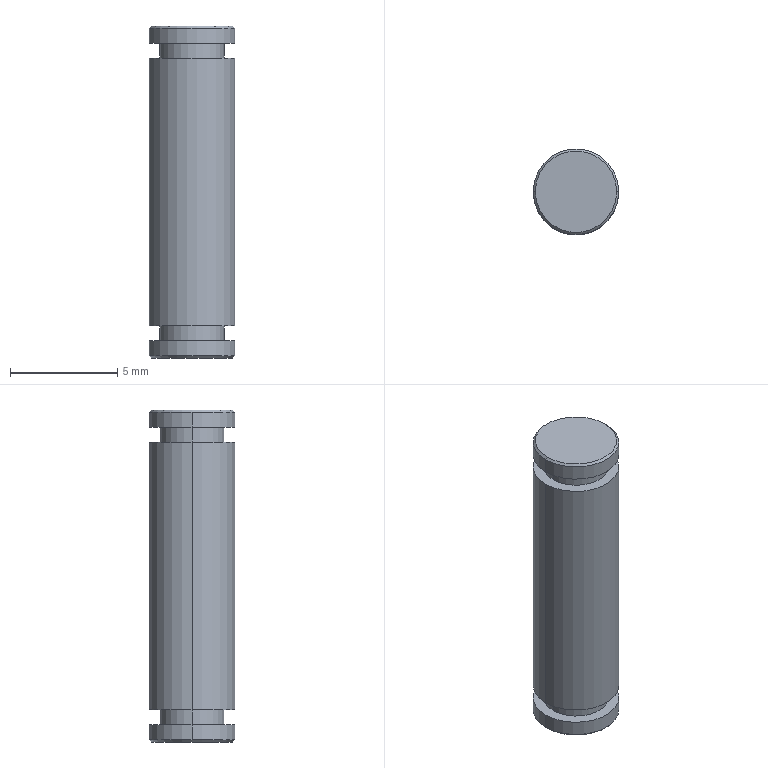Component | SolidWorks | JR-PL-JD-06ConnectingRodPin-1 | 1 solid | 20 faces | box 4 x 4 x 15.5 mm | volume 187 mm3 | cylinder 10 | plane 6 | cone 4 | commonest cylinder face diameters 4 x6 3 x4
build123d program:
from build123d import *

# Parameters (mm, degrees)
CHAMFER1_SIZE = 0.1


with BuildPart() as part:
    # Sketch1 → Revolve1 (revolve)
    with BuildSketch(Plane.XY, mode=Mode.PRIVATE) as revolve1_sk:
        Polygon((0, 0), (0, 2), (0.8, 2), (0.8, 1.5), (1.5, 1.5), (1.5, 2), (14, 2), (14, 1.5), (14.7, 1.5), (14.7, 2), (15.5, 2), (15.5, 0), align=None)
    revolve(revolve1_sk.sketch.rotate(Axis((0, 0, 0), (1, 0, 0)), 90), axis=Axis((0, 0, 0), (1, 0, 0)))

    # Chamfer1
    chamfer1_edges = [part.edges().sort_by_distance(p)[0] for p in [
        (0, 0, -2),
        (15.5, 0, -2),
    ]]
    chamfer(chamfer1_edges, length=CHAMFER1_SIZE)


solid = part.part

# Placed as in the assembly
solid = solid.moved(Location((16.506, 30.452, 78.52), (0, 90, 0)))
STEP:
#1=COLOUR_RGB('',0.7922,0.8196,0.9333);
#2=FILL_AREA_STYLE_COLOUR('',#1);
#3=FILL_AREA_STYLE('',(#2));
#4=SURFACE_STYLE_FILL_AREA(#3);
#5=SURFACE_SIDE_STYLE('',(#4));
#6=SURFACE_STYLE_USAGE(.BOTH.,#5);
#7=PRESENTATION_STYLE_ASSIGNMENT((#6));
#8=CARTESIAN_POINT('',(0.575,1.199,2.481));
#9=VERTEX_POINT('',#8);
#10=CARTESIAN_POINT('',(0.7246,1.199,2.481));
#11=VERTEX_POINT('',#10);
#12=CARTESIAN_POINT('',(0.6498,1.199,2.481));
#13=DIRECTION('',(0.,0.,-1.));
#14=DIRECTION('',(1.,0.,0.));
#15=AXIS2_PLACEMENT_3D('',#12,#13,#14);
#16=CIRCLE('',#15,0.0748);
#17=EDGE_CURVE('',#9,#11,#16,.T.);
#18=ORIENTED_EDGE('',*,*,#17,.F.);
#19=CARTESIAN_POINT('',(0.5711,1.199,2.485));
#20=VERTEX_POINT('',#19);
#21=CARTESIAN_POINT('',(0.575,1.199,2.481));
#22=DIRECTION('',(-0.7071,0.,0.7071));
#23=VECTOR('',#22,39.37);
#24=LINE('',#21,#23);
#25=EDGE_CURVE('',#9,#20,#24,.T.);
#26=ORIENTED_EDGE('',*,*,#25,.T.);
#27=CARTESIAN_POINT('',(0.7286,1.199,2.485));
#28=VERTEX_POINT('',#27);
#29=CARTESIAN_POINT('',(0.6498,1.199,2.485));
#30=DIRECTION('',(0.,0.,1.));
#31=DIRECTION('',(1.,0.,0.));
#32=AXIS2_PLACEMENT_3D('',#29,#30,#31);
#33=CIRCLE('',#32,0.07874);
#34=EDGE_CURVE('',#28,#20,#33,.T.);
#35=ORIENTED_EDGE('',*,*,#34,.F.);
#36=CARTESIAN_POINT('',(0.7246,1.199,2.481));
#37=DIRECTION('',(0.7071,0.,0.7071));
#38=VECTOR('',#37,39.37);
#39=LINE('',#36,#38);
#40=EDGE_CURVE('',#11,#28,#39,.T.);
#41=ORIENTED_EDGE('',*,*,#40,.F.);
#42=EDGE_LOOP('',(#18,#26,#35,#41));
#43=FACE_OUTER_BOUND('',#42,.T.);
#44=CARTESIAN_POINT('',(0.6498,1.199,2.481));
#45=DIRECTION('',(0.,0.,1.));
#46=DIRECTION('',(1.,0.,0.));
#47=AXIS2_PLACEMENT_3D('',#44,#45,#46);
#48=CONICAL_SURFACE('',#47,0.0748,0.7854);
#49=ADVANCED_FACE('',(#43),#48,.T.);
#50=CARTESIAN_POINT('',(0.7246,1.199,3.091));
#51=VERTEX_POINT('',#50);
#52=CARTESIAN_POINT('',(0.575,1.199,3.091));
#53=VERTEX_POINT('',#52);
#54=CARTESIAN_POINT('',(0.6498,1.199,3.091));
#55=DIRECTION('',(0.,0.,1.));
#56=DIRECTION('',(-1.,0.,0.));
#57=AXIS2_PLACEMENT_3D('',#54,#55,#56);
#58=CIRCLE('',#57,0.0748);
#59=EDGE_CURVE('',#51,#53,#58,.T.);
#60=ORIENTED_EDGE('',*,*,#59,.F.);
#61=CARTESIAN_POINT('',(0.7286,1.199,3.087));
#62=VERTEX_POINT('',#61);
#63=CARTESIAN_POINT('',(0.7286,1.199,3.087));
#64=DIRECTION('',(0.7071,0.,-0.7071));
#65=VECTOR('',#64,39.37);
#66=LINE('',#63,#65);
#67=EDGE_CURVE('',#51,#62,#66,.T.);
#68=ORIENTED_EDGE('',*,*,#67,.T.);
#69=CARTESIAN_POINT('',(0.5711,1.199,3.087));
#70=VERTEX_POINT('',#69);
#71=CARTESIAN_POINT('',(0.6498,1.199,3.087));
#72=DIRECTION('',(0.,0.,-1.));
#73=DIRECTION('',(-1.,0.,0.));
#74=AXIS2_PLACEMENT_3D('',#71,#72,#73);
#75=CIRCLE('',#74,0.07874);
#76=EDGE_CURVE('',#70,#62,#75,.T.);
#77=ORIENTED_EDGE('',*,*,#76,.F.);
#78=CARTESIAN_POINT('',(0.5711,1.199,3.087));
#79=DIRECTION('',(-0.7071,0.,-0.7071));
#80=VECTOR('',#79,39.37);
#81=LINE('',#78,#80);
#82=EDGE_CURVE('',#53,#70,#81,.T.);
#83=ORIENTED_EDGE('',*,*,#82,.F.);
#84=EDGE_LOOP('',(#60,#68,#77,#83));
#85=FACE_OUTER_BOUND('',#84,.T.);
#86=CARTESIAN_POINT('',(0.6498,1.199,3.087));
#87=DIRECTION('',(0.,0.,-1.));
#88=DIRECTION('',(-1.,0.,0.));
#89=AXIS2_PLACEMENT_3D('',#86,#87,#88);
#90=CONICAL_SURFACE('',#89,0.07874,0.7854);
#91=ADVANCED_FACE('',(#85),#90,.T.);
#92=ORIENTED_EDGE('',*,*,#76,.T.);
#93=CARTESIAN_POINT('',(0.7286,1.199,3.06));
#94=VERTEX_POINT('',#93);
#95=CARTESIAN_POINT('',(0.7286,1.199,2.481));
#96=DIRECTION('',(0.,0.,-1.));
#97=VECTOR('',#96,39.37);
#98=LINE('',#95,#97);
#99=EDGE_CURVE('',#62,#94,#98,.T.);
#100=ORIENTED_EDGE('',*,*,#99,.T.);
#101=CARTESIAN_POINT('',(0.5711,1.199,3.06));
#102=VERTEX_POINT('',#101);
#103=CARTESIAN_POINT('',(0.6498,1.199,3.06));
#104=DIRECTION('',(0.,0.,-1.));
#105=DIRECTION('',(-1.,0.,0.));
#106=AXIS2_PLACEMENT_3D('',#103,#104,#105);
#107=CIRCLE('',#106,0.07874);
#108=EDGE_CURVE('',#102,#94,#107,.T.);
#109=ORIENTED_EDGE('',*,*,#108,.F.);
#110=CARTESIAN_POINT('',(0.5711,1.199,2.481));
#111=DIRECTION('',(0.,0.,-1.));
#112=VECTOR('',#111,39.37);
#113=LINE('',#110,#112);
#114=EDGE_CURVE('',#70,#102,#113,.T.);
#115=ORIENTED_EDGE('',*,*,#114,.F.);
#116=EDGE_LOOP('',(#92,#100,#109,#115));
#117=FACE_OUTER_BOUND('',#116,.T.);
#118=CARTESIAN_POINT('',(0.6498,1.199,2.481));
#119=DIRECTION('',(0.,0.,-1.));
#120=DIRECTION('',(-1.,0.,0.));
#121=AXIS2_PLACEMENT_3D('',#118,#119,#120);
#122=CYLINDRICAL_SURFACE('',#121,0.07874);
#123=ADVANCED_FACE('',(#117),#122,.T.);
#124=CARTESIAN_POINT('',(0.5908,1.199,3.06));
#125=VERTEX_POINT('',#124);
#126=CARTESIAN_POINT('',(0.7089,1.199,3.06));
#127=VERTEX_POINT('',#126);
#128=CARTESIAN_POINT('',(0.6498,1.199,3.06));
#129=DIRECTION('',(0.,0.,-1.));
#130=DIRECTION('',(-1.,0.,0.));
#131=AXIS2_PLACEMENT_3D('',#128,#129,#130);
#132=CIRCLE('',#131,0.05906);
#133=EDGE_CURVE('',#125,#127,#132,.T.);
#134=ORIENTED_EDGE('',*,*,#133,.T.);
#135=CARTESIAN_POINT('',(0.7089,1.199,3.032));
#136=VERTEX_POINT('',#135);
#137=CARTESIAN_POINT('',(0.7089,1.199,2.481));
#138=DIRECTION('',(0.,0.,-1.));
#139=VECTOR('',#138,39.37);
#140=LINE('',#137,#139);
#141=EDGE_CURVE('',#127,#136,#140,.T.);
#142=ORIENTED_EDGE('',*,*,#141,.T.);
#143=CARTESIAN_POINT('',(0.5908,1.199,3.032));
#144=VERTEX_POINT('',#143);
#145=CARTESIAN_POINT('',(0.6498,1.199,3.032));
#146=DIRECTION('',(0.,0.,-1.));
#147=DIRECTION('',(-1.,0.,0.));
#148=AXIS2_PLACEMENT_3D('',#145,#146,#147);
#149=CIRCLE('',#148,0.05906);
#150=EDGE_CURVE('',#144,#136,#149,.T.);
#151=ORIENTED_EDGE('',*,*,#150,.F.);
#152=CARTESIAN_POINT('',(0.5908,1.199,2.481));
#153=DIRECTION('',(0.,0.,-1.));
#154=VECTOR('',#153,39.37);
#155=LINE('',#152,#154);
#156=EDGE_CURVE('',#125,#144,#155,.T.);
#157=ORIENTED_EDGE('',*,*,#156,.F.);
#158=EDGE_LOOP('',(#134,#142,#151,#157));
#159=FACE_OUTER_BOUND('',#158,.T.);
#160=CARTESIAN_POINT('',(0.6498,1.199,2.481));
#161=DIRECTION('',(0.,0.,-1.));
#162=DIRECTION('',(-1.,0.,0.));
#163=AXIS2_PLACEMENT_3D('',#160,#161,#162);
#164=CYLINDRICAL_SURFACE('',#163,0.05906);
#165=ADVANCED_FACE('',(#159),#164,.T.);
#166=CARTESIAN_POINT('',(0.5711,1.199,3.032));
#167=VERTEX_POINT('',#166);
#168=CARTESIAN_POINT('',(0.7286,1.199,3.032));
#169=VERTEX_POINT('',#168);
#170=CARTESIAN_POINT('',(0.6498,1.199,3.032));
#171=DIRECTION('',(0.,0.,-1.));
#172=DIRECTION('',(-1.,0.,0.));
#173=AXIS2_PLACEMENT_3D('',#170,#171,#172);
#174=CIRCLE('',#173,0.07874);
#175=EDGE_CURVE('',#167,#169,#174,.T.);
#176=ORIENTED_EDGE('',*,*,#175,.T.);
#177=CARTESIAN_POINT('',(0.7286,1.199,2.54));
#178=VERTEX_POINT('',#177);
#179=CARTESIAN_POINT('',(0.7286,1.199,2.481));
#180=DIRECTION('',(0.,0.,-1.));
#181=VECTOR('',#180,39.37);
#182=LINE('',#179,#181);
#183=EDGE_CURVE('',#169,#178,#182,.T.);
#184=ORIENTED_EDGE('',*,*,#183,.T.);
#185=CARTESIAN_POINT('',(0.5711,1.199,2.54));
#186=VERTEX_POINT('',#185);
#187=CARTESIAN_POINT('',(0.6498,1.199,2.54));
#188=DIRECTION('',(0.,0.,-1.));
#189=DIRECTION('',(-1.,0.,0.));
#190=AXIS2_PLACEMENT_3D('',#187,#188,#189);
#191=CIRCLE('',#190,0.07874);
#192=EDGE_CURVE('',#186,#178,#191,.T.);
#193=ORIENTED_EDGE('',*,*,#192,.F.);
#194=CARTESIAN_POINT('',(0.5711,1.199,2.481));
#195=DIRECTION('',(0.,0.,-1.));
#196=VECTOR('',#195,39.37);
#197=LINE('',#194,#196);
#198=EDGE_CURVE('',#167,#186,#197,.T.);
#199=ORIENTED_EDGE('',*,*,#198,.F.);
#200=EDGE_LOOP('',(#176,#184,#193,#199));
#201=FACE_OUTER_BOUND('',#200,.T.);
#202=CARTESIAN_POINT('',(0.6498,1.199,2.481));
#203=DIRECTION('',(0.,0.,-1.));
#204=DIRECTION('',(-1.,0.,0.));
#205=AXIS2_PLACEMENT_3D('',#202,#203,#204);
#206=CYLINDRICAL_SURFACE('',#205,0.07874);
#207=ADVANCED_FACE('',(#201),#206,.T.);
#208=CARTESIAN_POINT('',(0.5908,1.199,2.54));
#209=VERTEX_POINT('',#208);
#210=CARTESIAN_POINT('',(0.7089,1.199,2.54));
#211=VERTEX_POINT('',#210);
#212=CARTESIAN_POINT('',(0.6498,1.199,2.54));
#213=DIRECTION('',(0.,0.,-1.));
#214=DIRECTION('',(-1.,0.,0.));
#215=AXIS2_PLACEMENT_3D('',#212,#213,#214);
#216=CIRCLE('',#215,0.05906);
#217=EDGE_CURVE('',#209,#211,#216,.T.);
#218=ORIENTED_EDGE('',*,*,#217,.T.);
#219=CARTESIAN_POINT('',(0.7089,1.199,2.513));
#220=VERTEX_POINT('',#219);
#221=CARTESIAN_POINT('',(0.7089,1.199,2.481));
#222=DIRECTION('',(0.,0.,-1.));
#223=VECTOR('',#222,39.37);
#224=LINE('',#221,#223);
#225=EDGE_CURVE('',#211,#220,#224,.T.);
#226=ORIENTED_EDGE('',*,*,#225,.T.);
#227=CARTESIAN_POINT('',(0.5908,1.199,2.513));
#228=VERTEX_POINT('',#227);
#229=CARTESIAN_POINT('',(0.6498,1.199,2.513));
#230=DIRECTION('',(0.,0.,-1.));
#231=DIRECTION('',(-1.,0.,0.));
#232=AXIS2_PLACEMENT_3D('',#229,#230,#231);
#233=CIRCLE('',#232,0.05906);
#234=EDGE_CURVE('',#228,#220,#233,.T.);
#235=ORIENTED_EDGE('',*,*,#234,.F.);
#236=CARTESIAN_POINT('',(0.5908,1.199,2.481));
#237=DIRECTION('',(0.,0.,-1.));
#238=VECTOR('',#237,39.37);
#239=LINE('',#236,#238);
#240=EDGE_CURVE('',#209,#228,#239,.T.);
#241=ORIENTED_EDGE('',*,*,#240,.F.);
#242=EDGE_LOOP('',(#218,#226,#235,#241));
#243=FACE_OUTER_BOUND('',#242,.T.);
#244=CARTESIAN_POINT('',(0.6498,1.199,2.481));
#245=DIRECTION('',(0.,0.,-1.));
#246=DIRECTION('',(-1.,0.,0.));
#247=AXIS2_PLACEMENT_3D('',#244,#245,#246);
#248=CYLINDRICAL_SURFACE('',#247,0.05906);
#249=ADVANCED_FACE('',(#243),#248,.T.);
#250=CARTESIAN_POINT('',(0.5711,1.199,2.513));
#251=VERTEX_POINT('',#250);
#252=CARTESIAN_POINT('',(0.7286,1.199,2.513));
#253=VERTEX_POINT('',#252);
#254=CARTESIAN_POINT('',(0.6498,1.199,2.513));
#255=DIRECTION('',(0.,0.,-1.));
#256=DIRECTION('',(-1.,0.,0.));
#257=AXIS2_PLACEMENT_3D('',#254,#255,#256);
#258=CIRCLE('',#257,0.07874);
#259=EDGE_CURVE('',#251,#253,#258,.T.);
#260=ORIENTED_EDGE('',*,*,#259,.T.);
#261=CARTESIAN_POINT('',(0.7286,1.199,2.481));
#262=DIRECTION('',(0.,0.,-1.));
#263=VECTOR('',#262,39.37);
#264=LINE('',#261,#263);
#265=EDGE_CURVE('',#253,#28,#264,.T.);
#266=ORIENTED_EDGE('',*,*,#265,.T.);
#267=ORIENTED_EDGE('',*,*,#34,.T.);
#268=CARTESIAN_POINT('',(0.5711,1.199,2.481));
#269=DIRECTION('',(0.,0.,-1.));
#270=VECTOR('',#269,39.37);
#271=LINE('',#268,#270);
#272=EDGE_CURVE('',#251,#20,#271,.T.);
#273=ORIENTED_EDGE('',*,*,#272,.F.);
#274=EDGE_LOOP('',(#260,#266,#267,#273));
#275=FACE_OUTER_BOUND('',#274,.T.);
#276=CARTESIAN_POINT('',(0.6498,1.199,2.481));
#277=DIRECTION('',(0.,0.,-1.));
#278=DIRECTION('',(-1.,0.,0.));
#279=AXIS2_PLACEMENT_3D('',#276,#277,#278);
#280=CYLINDRICAL_SURFACE('',#279,0.07874);
#281=ADVANCED_FACE('',(#275),#280,.T.);
#282=CARTESIAN_POINT('',(0.6498,1.199,2.481));
#283=DIRECTION('',(0.,0.,-1.));
#284=DIRECTION('',(1.,0.,0.));
#285=AXIS2_PLACEMENT_3D('',#282,#283,#284);
#286=CIRCLE('',#285,0.0748);
#287=EDGE_CURVE('',#11,#9,#286,.T.);
#288=ORIENTED_EDGE('',*,*,#287,.T.);
#289=ORIENTED_EDGE('',*,*,#17,.T.);
#290=EDGE_LOOP('',(#288,#289));
#291=FACE_OUTER_BOUND('',#290,.T.);
#292=CARTESIAN_POINT('',(0.6498,1.199,2.481));
#293=DIRECTION('',(0.,0.,1.));
#294=DIRECTION('',(1.,0.,0.));
#295=AXIS2_PLACEMENT_3D('',#292,#293,#294);
#296=PLANE('',#295);
#297=ADVANCED_FACE('',(#291),#296,.F.);
#298=ORIENTED_EDGE('',*,*,#265,.F.);
#299=CARTESIAN_POINT('',(0.6498,1.199,2.513));
#300=DIRECTION('',(0.,0.,-1.));
#301=DIRECTION('',(-1.,0.,0.));
#302=AXIS2_PLACEMENT_3D('',#299,#300,#301);
#303=CIRCLE('',#302,0.07874);
#304=EDGE_CURVE('',#253,#251,#303,.T.);
#305=ORIENTED_EDGE('',*,*,#304,.T.);
#306=ORIENTED_EDGE('',*,*,#272,.T.);
#307=CARTESIAN_POINT('',(0.6498,1.199,2.485));
#308=DIRECTION('',(0.,0.,1.));
#309=DIRECTION('',(1.,0.,0.));
#310=AXIS2_PLACEMENT_3D('',#307,#308,#309);
#311=CIRCLE('',#310,0.07874);
#312=EDGE_CURVE('',#20,#28,#311,.T.);
#313=ORIENTED_EDGE('',*,*,#312,.T.);
#314=EDGE_LOOP('',(#298,#305,#306,#313));
#315=FACE_OUTER_BOUND('',#314,.T.);
#316=CARTESIAN_POINT('',(0.6498,1.199,2.481));
#317=DIRECTION('',(0.,0.,-1.));
#318=DIRECTION('',(-1.,0.,0.));
#319=AXIS2_PLACEMENT_3D('',#316,#317,#318);
#320=CYLINDRICAL_SURFACE('',#319,0.07874);
#321=ADVANCED_FACE('',(#315),#320,.T.);
#322=ORIENTED_EDGE('',*,*,#259,.F.);
#323=ORIENTED_EDGE('',*,*,#304,.F.);
#324=EDGE_LOOP('',(#322,#323));
#325=FACE_OUTER_BOUND('',#324,.T.);
#326=ORIENTED_EDGE('',*,*,#234,.T.);
#327=CARTESIAN_POINT('',(0.6498,1.199,2.513));
#328=DIRECTION('',(0.,0.,-1.));
#329=DIRECTION('',(-1.,0.,0.));
#330=AXIS2_PLACEMENT_3D('',#327,#328,#329);
#331=CIRCLE('',#330,0.05906);
#332=EDGE_CURVE('',#220,#228,#331,.T.);
#333=ORIENTED_EDGE('',*,*,#332,.T.);
#334=EDGE_LOOP('',(#326,#333));
#335=FACE_BOUND('',#334,.T.);
#336=CARTESIAN_POINT('',(0.6498,1.278,2.513));
#337=DIRECTION('',(0.,0.,-1.));
#338=DIRECTION('',(-1.,0.,0.));
#339=AXIS2_PLACEMENT_3D('',#336,#337,#338);
#340=PLANE('',#339);
#341=ADVANCED_FACE('',(#325,#335),#340,.F.);
#342=ORIENTED_EDGE('',*,*,#225,.F.);
#343=CARTESIAN_POINT('',(0.6498,1.199,2.54));
#344=DIRECTION('',(0.,0.,-1.));
#345=DIRECTION('',(-1.,0.,0.));
#346=AXIS2_PLACEMENT_3D('',#343,#344,#345);
#347=CIRCLE('',#346,0.05906);
#348=EDGE_CURVE('',#211,#209,#347,.T.);
#349=ORIENTED_EDGE('',*,*,#348,.T.);
#350=ORIENTED_EDGE('',*,*,#240,.T.);
#351=ORIENTED_EDGE('',*,*,#332,.F.);
#352=EDGE_LOOP('',(#342,#349,#350,#351));
#353=FACE_OUTER_BOUND('',#352,.T.);
#354=CARTESIAN_POINT('',(0.6498,1.199,2.481));
#355=DIRECTION('',(0.,0.,-1.));
#356=DIRECTION('',(-1.,0.,0.));
#357=AXIS2_PLACEMENT_3D('',#354,#355,#356);
#358=CYLINDRICAL_SURFACE('',#357,0.05906);
#359=ADVANCED_FACE('',(#353),#358,.T.);
#360=ORIENTED_EDGE('',*,*,#217,.F.);
#361=ORIENTED_EDGE('',*,*,#348,.F.);
#362=EDGE_LOOP('',(#360,#361));
#363=FACE_BOUND('',#362,.T.);
#364=ORIENTED_EDGE('',*,*,#192,.T.);
#365=CARTESIAN_POINT('',(0.6498,1.199,2.54));
#366=DIRECTION('',(0.,0.,-1.));
#367=DIRECTION('',(-1.,0.,0.));
#368=AXIS2_PLACEMENT_3D('',#365,#366,#367);
#369=CIRCLE('',#368,0.07874);
#370=EDGE_CURVE('',#178,#186,#369,.T.);
#371=ORIENTED_EDGE('',*,*,#370,.T.);
#372=EDGE_LOOP('',(#364,#371));
#373=FACE_OUTER_BOUND('',#372,.T.);
#374=CARTESIAN_POINT('',(0.6498,1.258,2.54));
#375=DIRECTION('',(0.,0.,1.));
#376=DIRECTION('',(1.,0.,0.));
#377=AXIS2_PLACEMENT_3D('',#374,#375,#376);
#378=PLANE('',#377);
#379=ADVANCED_FACE('',(#363,#373),#378,.F.);
#380=ORIENTED_EDGE('',*,*,#183,.F.);
#381=CARTESIAN_POINT('',(0.6498,1.199,3.032));
#382=DIRECTION('',(0.,0.,-1.));
#383=DIRECTION('',(-1.,0.,0.));
#384=AXIS2_PLACEMENT_3D('',#381,#382,#383);
#385=CIRCLE('',#384,0.07874);
#386=EDGE_CURVE('',#169,#167,#385,.T.);
#387=ORIENTED_EDGE('',*,*,#386,.T.);
#388=ORIENTED_EDGE('',*,*,#198,.T.);
#389=ORIENTED_EDGE('',*,*,#370,.F.);
#390=EDGE_LOOP('',(#380,#387,#388,#389));
#391=FACE_OUTER_BOUND('',#390,.T.);
#392=CARTESIAN_POINT('',(0.6498,1.199,2.481));
#393=DIRECTION('',(0.,0.,-1.));
#394=DIRECTION('',(-1.,0.,0.));
#395=AXIS2_PLACEMENT_3D('',#392,#393,#394);
#396=CYLINDRICAL_SURFACE('',#395,0.07874);
#397=ADVANCED_FACE('',(#391),#396,.T.);
#398=ORIENTED_EDGE('',*,*,#175,.F.);
#399=ORIENTED_EDGE('',*,*,#386,.F.);
#400=EDGE_LOOP('',(#398,#399));
#401=FACE_OUTER_BOUND('',#400,.T.);
#402=ORIENTED_EDGE('',*,*,#150,.T.);
#403=CARTESIAN_POINT('',(0.6498,1.199,3.032));
#404=DIRECTION('',(0.,0.,-1.));
#405=DIRECTION('',(-1.,0.,0.));
#406=AXIS2_PLACEMENT_3D('',#403,#404,#405);
#407=CIRCLE('',#406,0.05906);
#408=EDGE_CURVE('',#136,#144,#407,.T.);
#409=ORIENTED_EDGE('',*,*,#408,.T.);
#410=EDGE_LOOP('',(#402,#409));
#411=FACE_BOUND('',#410,.T.);
#412=CARTESIAN_POINT('',(0.6498,1.258,3.032));
#413=DIRECTION('',(0.,0.,-1.));
#414=DIRECTION('',(-1.,0.,0.));
#415=AXIS2_PLACEMENT_3D('',#412,#413,#414);
#416=PLANE('',#415);
#417=ADVANCED_FACE('',(#401,#411),#416,.F.);
#418=ORIENTED_EDGE('',*,*,#141,.F.);
#419=CARTESIAN_POINT('',(0.6498,1.199,3.06));
#420=DIRECTION('',(0.,0.,-1.));
#421=DIRECTION('',(-1.,0.,0.));
#422=AXIS2_PLACEMENT_3D('',#419,#420,#421);
#423=CIRCLE('',#422,0.05906);
#424=EDGE_CURVE('',#127,#125,#423,.T.);
#425=ORIENTED_EDGE('',*,*,#424,.T.);
#426=ORIENTED_EDGE('',*,*,#156,.T.);
#427=ORIENTED_EDGE('',*,*,#408,.F.);
#428=EDGE_LOOP('',(#418,#425,#426,#427));
#429=FACE_OUTER_BOUND('',#428,.T.);
#430=CARTESIAN_POINT('',(0.6498,1.199,2.481));
#431=DIRECTION('',(0.,0.,-1.));
#432=DIRECTION('',(-1.,0.,0.));
#433=AXIS2_PLACEMENT_3D('',#430,#431,#432);
#434=CYLINDRICAL_SURFACE('',#433,0.05906);
#435=ADVANCED_FACE('',(#429),#434,.T.);
#436=ORIENTED_EDGE('',*,*,#133,.F.);
#437=ORIENTED_EDGE('',*,*,#424,.F.);
#438=EDGE_LOOP('',(#436,#437));
#439=FACE_BOUND('',#438,.T.);
#440=ORIENTED_EDGE('',*,*,#108,.T.);
#441=CARTESIAN_POINT('',(0.6498,1.199,3.06));
#442=DIRECTION('',(0.,0.,-1.));
#443=DIRECTION('',(-1.,0.,0.));
#444=AXIS2_PLACEMENT_3D('',#441,#442,#443);
#445=CIRCLE('',#444,0.07874);
#446=EDGE_CURVE('',#94,#102,#445,.T.);
#447=ORIENTED_EDGE('',*,*,#446,.T.);
#448=EDGE_LOOP('',(#440,#447));
#449=FACE_OUTER_BOUND('',#448,.T.);
#450=CARTESIAN_POINT('',(0.6498,1.278,3.06));
#451=DIRECTION('',(0.,0.,1.));
#452=DIRECTION('',(1.,0.,0.));
#453=AXIS2_PLACEMENT_3D('',#450,#451,#452);
#454=PLANE('',#453);
#455=ADVANCED_FACE('',(#439,#449),#454,.F.);
#456=ORIENTED_EDGE('',*,*,#99,.F.);
#457=CARTESIAN_POINT('',(0.6498,1.199,3.087));
#458=DIRECTION('',(0.,0.,-1.));
#459=DIRECTION('',(-1.,0.,0.));
#460=AXIS2_PLACEMENT_3D('',#457,#458,#459);
#461=CIRCLE('',#460,0.07874);
#462=EDGE_CURVE('',#62,#70,#461,.T.);
#463=ORIENTED_EDGE('',*,*,#462,.T.);
#464=ORIENTED_EDGE('',*,*,#114,.T.);
#465=ORIENTED_EDGE('',*,*,#446,.F.);
#466=EDGE_LOOP('',(#456,#463,#464,#465));
#467=FACE_OUTER_BOUND('',#466,.T.);
#468=CARTESIAN_POINT('',(0.6498,1.199,2.481));
#469=DIRECTION('',(0.,0.,-1.));
#470=DIRECTION('',(-1.,0.,0.));
#471=AXIS2_PLACEMENT_3D('',#468,#469,#470);
#472=CYLINDRICAL_SURFACE('',#471,0.07874);
#473=ADVANCED_FACE('',(#467),#472,.T.);
#474=CARTESIAN_POINT('',(0.6498,1.199,3.091));
#475=DIRECTION('',(0.,0.,1.));
#476=DIRECTION('',(-1.,0.,0.));
#477=AXIS2_PLACEMENT_3D('',#474,#475,#476);
#478=CIRCLE('',#477,0.0748);
#479=EDGE_CURVE('',#53,#51,#478,.T.);
#480=ORIENTED_EDGE('',*,*,#479,.T.);
#481=ORIENTED_EDGE('',*,*,#59,.T.);
#482=EDGE_LOOP('',(#480,#481));
#483=FACE_OUTER_BOUND('',#482,.T.);
#484=CARTESIAN_POINT('',(0.6498,1.199,3.091));
#485=DIRECTION('',(0.,0.,-1.));
#486=DIRECTION('',(-1.,0.,0.));
#487=AXIS2_PLACEMENT_3D('',#484,#485,#486);
#488=PLANE('',#487);
#489=ADVANCED_FACE('',(#483),#488,.F.);
#490=ORIENTED_EDGE('',*,*,#67,.F.);
#491=ORIENTED_EDGE('',*,*,#479,.F.);
#492=ORIENTED_EDGE('',*,*,#82,.T.);
#493=ORIENTED_EDGE('',*,*,#462,.F.);
#494=EDGE_LOOP('',(#490,#491,#492,#493));
#495=FACE_OUTER_BOUND('',#494,.T.);
#496=CARTESIAN_POINT('',(0.6498,1.199,3.087));
#497=DIRECTION('',(0.,0.,-1.));
#498=DIRECTION('',(-1.,0.,0.));
#499=AXIS2_PLACEMENT_3D('',#496,#497,#498);
#500=CONICAL_SURFACE('',#499,0.07874,0.7854);
#501=ADVANCED_FACE('',(#495),#500,.T.);
#502=ORIENTED_EDGE('',*,*,#25,.F.);
#503=ORIENTED_EDGE('',*,*,#287,.F.);
#504=ORIENTED_EDGE('',*,*,#40,.T.);
#505=ORIENTED_EDGE('',*,*,#312,.F.);
#506=EDGE_LOOP('',(#502,#503,#504,#505));
#507=FACE_OUTER_BOUND('',#506,.T.);
#508=CARTESIAN_POINT('',(0.6498,1.199,2.481));
#509=DIRECTION('',(0.,0.,1.));
#510=DIRECTION('',(1.,0.,0.));
#511=AXIS2_PLACEMENT_3D('',#508,#509,#510);
#512=CONICAL_SURFACE('',#511,0.0748,0.7854);
#513=ADVANCED_FACE('',(#507),#512,.T.);
#514=CLOSED_SHELL('',(#49,#91,#123,#165,#207,#249,#281,#297,#321,#341,#359,#379,#397,#417,#435,#455,#473,#489,#501,#513));
#515=MANIFOLD_SOLID_BREP('',#514);
#516=STYLED_ITEM('',(#7),#515);
#517=PRESENTATION_LAYER_ASSIGNMENT('','',(#516));
#518=(LENGTH_UNIT()NAMED_UNIT(*)SI_UNIT($,.METRE.));
#519=LENGTH_MEASURE_WITH_UNIT(LENGTH_MEASURE(0.0254),#518);
#520=DIMENSIONAL_EXPONENTS(1.,0.,0.,0.,0.,0.,0.);
#521=(CONVERSION_BASED_UNIT('',#519)LENGTH_UNIT()NAMED_UNIT(#520));
#522=UNCERTAINTY_MEASURE_WITH_UNIT(LENGTH_MEASURE(0.00001),#521,'','');
#523=(NAMED_UNIT(*)PLANE_ANGLE_UNIT()SI_UNIT($,.RADIAN.));
#524=(NAMED_UNIT(*)SI_UNIT($,.STERADIAN.)SOLID_ANGLE_UNIT());
#525=(GEOMETRIC_REPRESENTATION_CONTEXT(3)GLOBAL_UNCERTAINTY_ASSIGNED_CONTEXT((#522))GLOBAL_UNIT_ASSIGNED_CONTEXT((#521,#523,#524))REPRESENTATION_CONTEXT('',''));
#526=MECHANICAL_DESIGN_GEOMETRIC_PRESENTATION_REPRESENTATION('',(#516),#525);
#527=CARTESIAN_POINT('',(0.,0.,0.));
#528=DIRECTION('',(0.,0.,1.));
#529=DIRECTION('',(1.,0.,0.));
#530=AXIS2_PLACEMENT_3D('',#527,#528,#529);
#531=(LENGTH_UNIT()NAMED_UNIT(*)SI_UNIT($,.METRE.));
#532=LENGTH_MEASURE_WITH_UNIT(LENGTH_MEASURE(0.0254),#531);
#533=DIMENSIONAL_EXPONENTS(1.,0.,0.,0.,0.,0.,0.);
#534=(CONVERSION_BASED_UNIT('',#532)LENGTH_UNIT()NAMED_UNIT(#533));
#535=UNCERTAINTY_MEASURE_WITH_UNIT(LENGTH_MEASURE(0.00001),#534,'','');
#536=(NAMED_UNIT(*)PLANE_ANGLE_UNIT()SI_UNIT($,.RADIAN.));
#537=(NAMED_UNIT(*)SI_UNIT($,.STERADIAN.)SOLID_ANGLE_UNIT());
#538=(GEOMETRIC_REPRESENTATION_CONTEXT(3)GLOBAL_UNCERTAINTY_ASSIGNED_CONTEXT((#535))GLOBAL_UNIT_ASSIGNED_CONTEXT((#534,#536,#537))REPRESENTATION_CONTEXT('',''));
#539=ADVANCED_BREP_SHAPE_REPRESENTATION('',(#515,#530),#538);